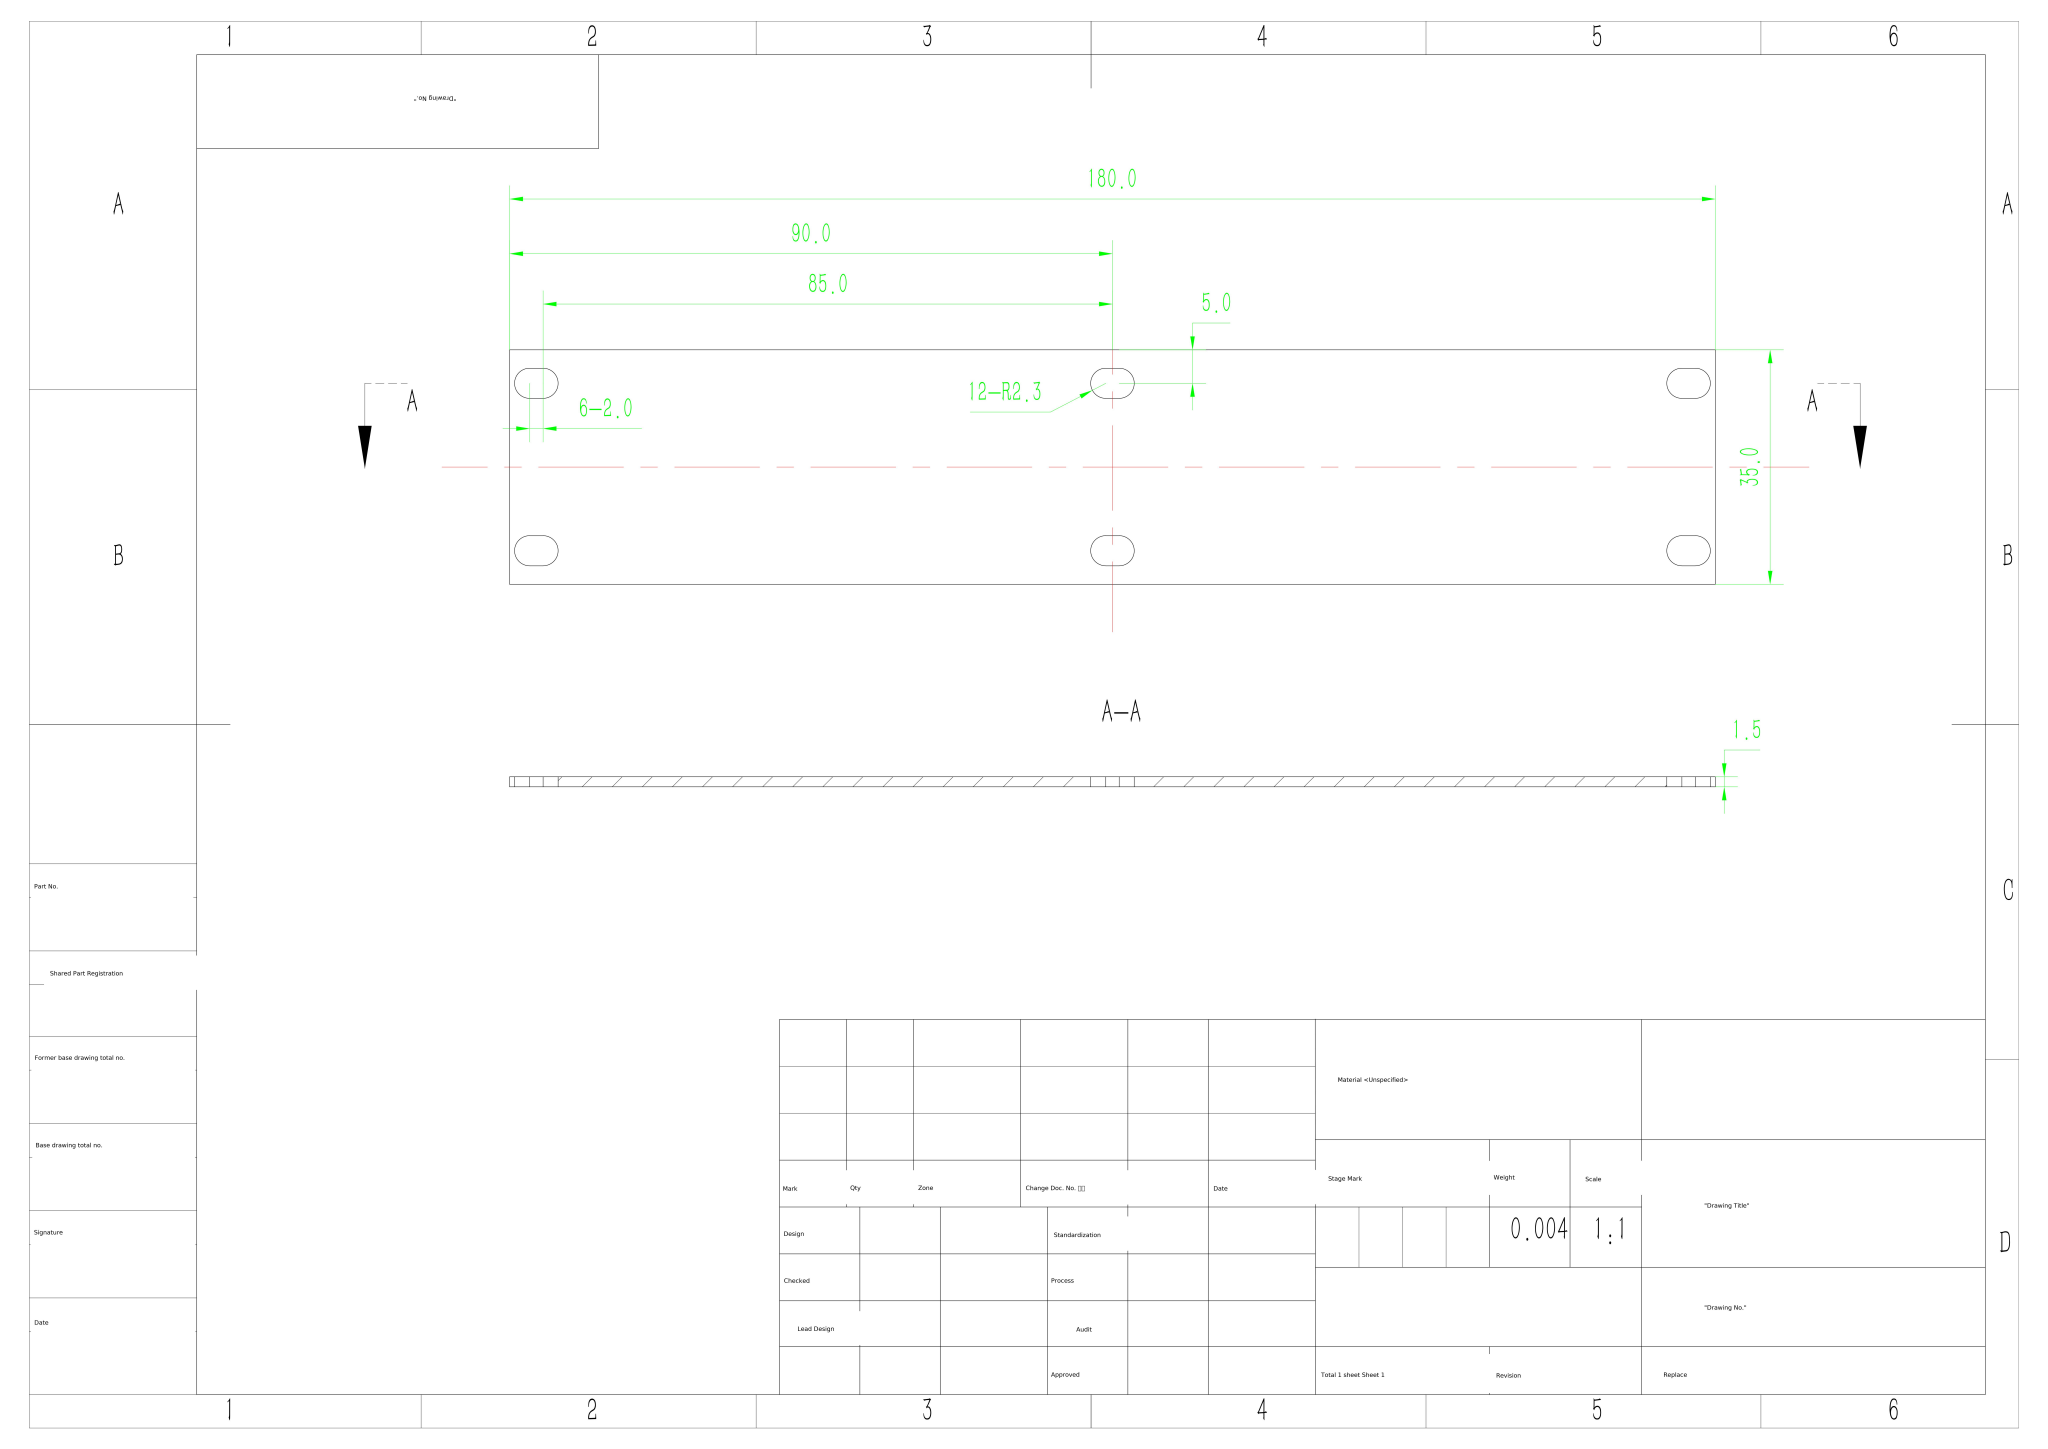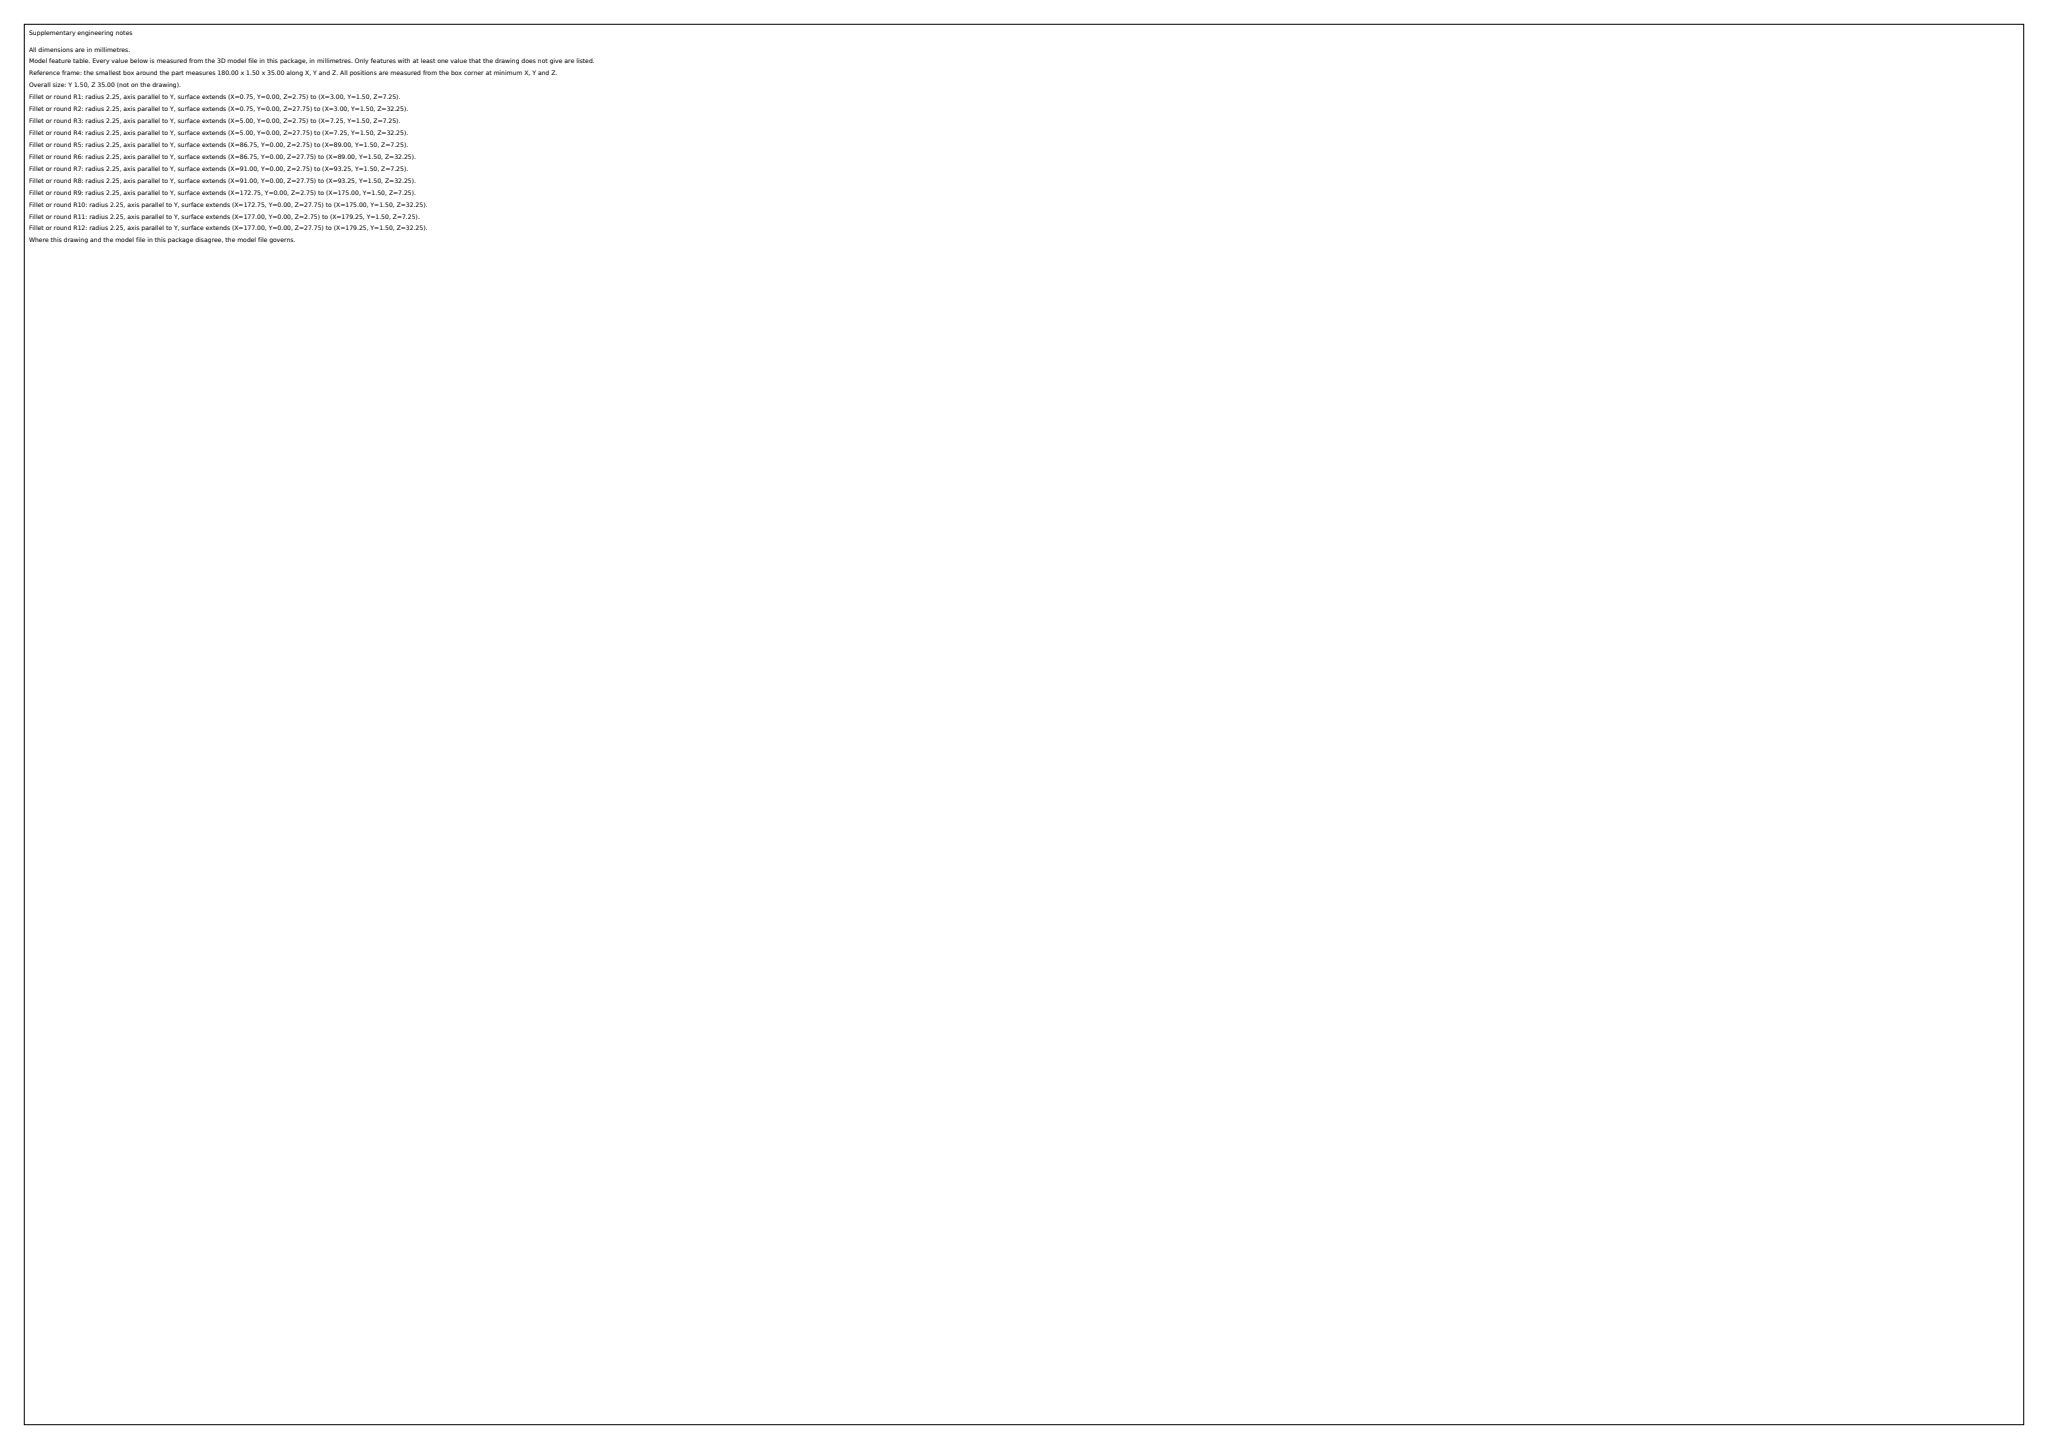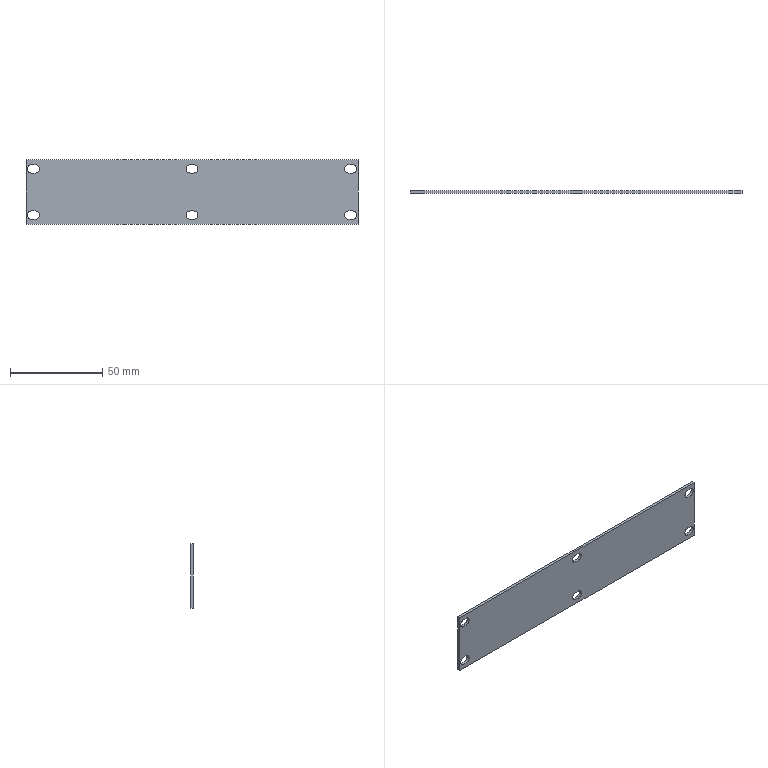Part | SolidWorks | mm | material <Unspecified> | 1 solid | 30 faces | box 180 x 1.5 x 35 mm | volume 9226 mm3 | plane 18 | cylinder 12 | commonest cylinder face diameters 4.5 x12
build123d program:
from build123d import *

# Parameters (mm, degrees)
SKETCH1_W           = 180
SKETCH1_H           = 35
BOSS_EXTRUDE1_DEPTH = 1.5
CUT_EXTRUDE1_DEPTH  = 92.698


with BuildPart() as part:
    # Sketch1 → Boss-Extrude1 (new body)
    with BuildSketch(Plane(origin=(0, 0, 0), x_dir=(1, 0, 0), z_dir=(0, 1, 0))):
        Rectangle(SKETCH1_W, SKETCH1_H)
    extrude(amount=BOSS_EXTRUDE1_DEPTH)

    # Sketch2 → Cut-Extrude1 (cut, through all)
    with BuildSketch(Plane(origin=(0, 1.5, 0), x_dir=(1, 0, 0), z_dir=(0, 1, 0))):
        with BuildLine():
            Line((-1, 14.75), (1, 14.75))
            ThreePointArc((1, 14.75), (3.25, 12.5), (1, 10.25))
            Line((1, 10.25), (-1, 10.25))
            ThreePointArc((-1, 10.25), (-3.25, 12.5), (-1, 14.75))
        make_face()
        with BuildLine():
            Line((85, 14.75), (87, 14.75))
            ThreePointArc((87, 14.75), (89.25, 12.5), (87, 10.25))
            Line((87, 10.25), (85, 10.25))
            ThreePointArc((85, 10.25), (82.75, 12.5), (85, 14.75))
        make_face()
        with BuildLine():
            Line((-85, 10.25), (-87, 10.25))
            ThreePointArc((-87, 10.25), (-89.25, 12.5), (-87, 14.75))
            Line((-87, 14.75), (-85, 14.75))
            ThreePointArc((-85, 14.75), (-82.75, 12.5), (-85, 10.25))
        make_face()
        with BuildLine():
            Line((-85, -10.25), (-87, -10.25))
            ThreePointArc((-87, -10.25), (-89.25, -12.5), (-87, -14.75))
            Line((-87, -14.75), (-85, -14.75))
            ThreePointArc((-85, -14.75), (-82.75, -12.5), (-85, -10.25))
        make_face()
        with BuildLine():
            Line((-1, -14.75), (1, -14.75))
            ThreePointArc((1, -14.75), (3.25, -12.5), (1, -10.25))
            Line((1, -10.25), (-1, -10.25))
            ThreePointArc((-1, -10.25), (-3.25, -12.5), (-1, -14.75))
        make_face()
        with BuildLine():
            Line((85, -14.75), (87, -14.75))
            ThreePointArc((87, -14.75), (89.25, -12.5), (87, -10.25))
            Line((87, -10.25), (85, -10.25))
            ThreePointArc((85, -10.25), (82.75, -12.5), (85, -14.75))
        make_face()
    extrude(amount=-CUT_EXTRUDE1_DEPTH, mode=Mode.SUBTRACT)


solid = part.part